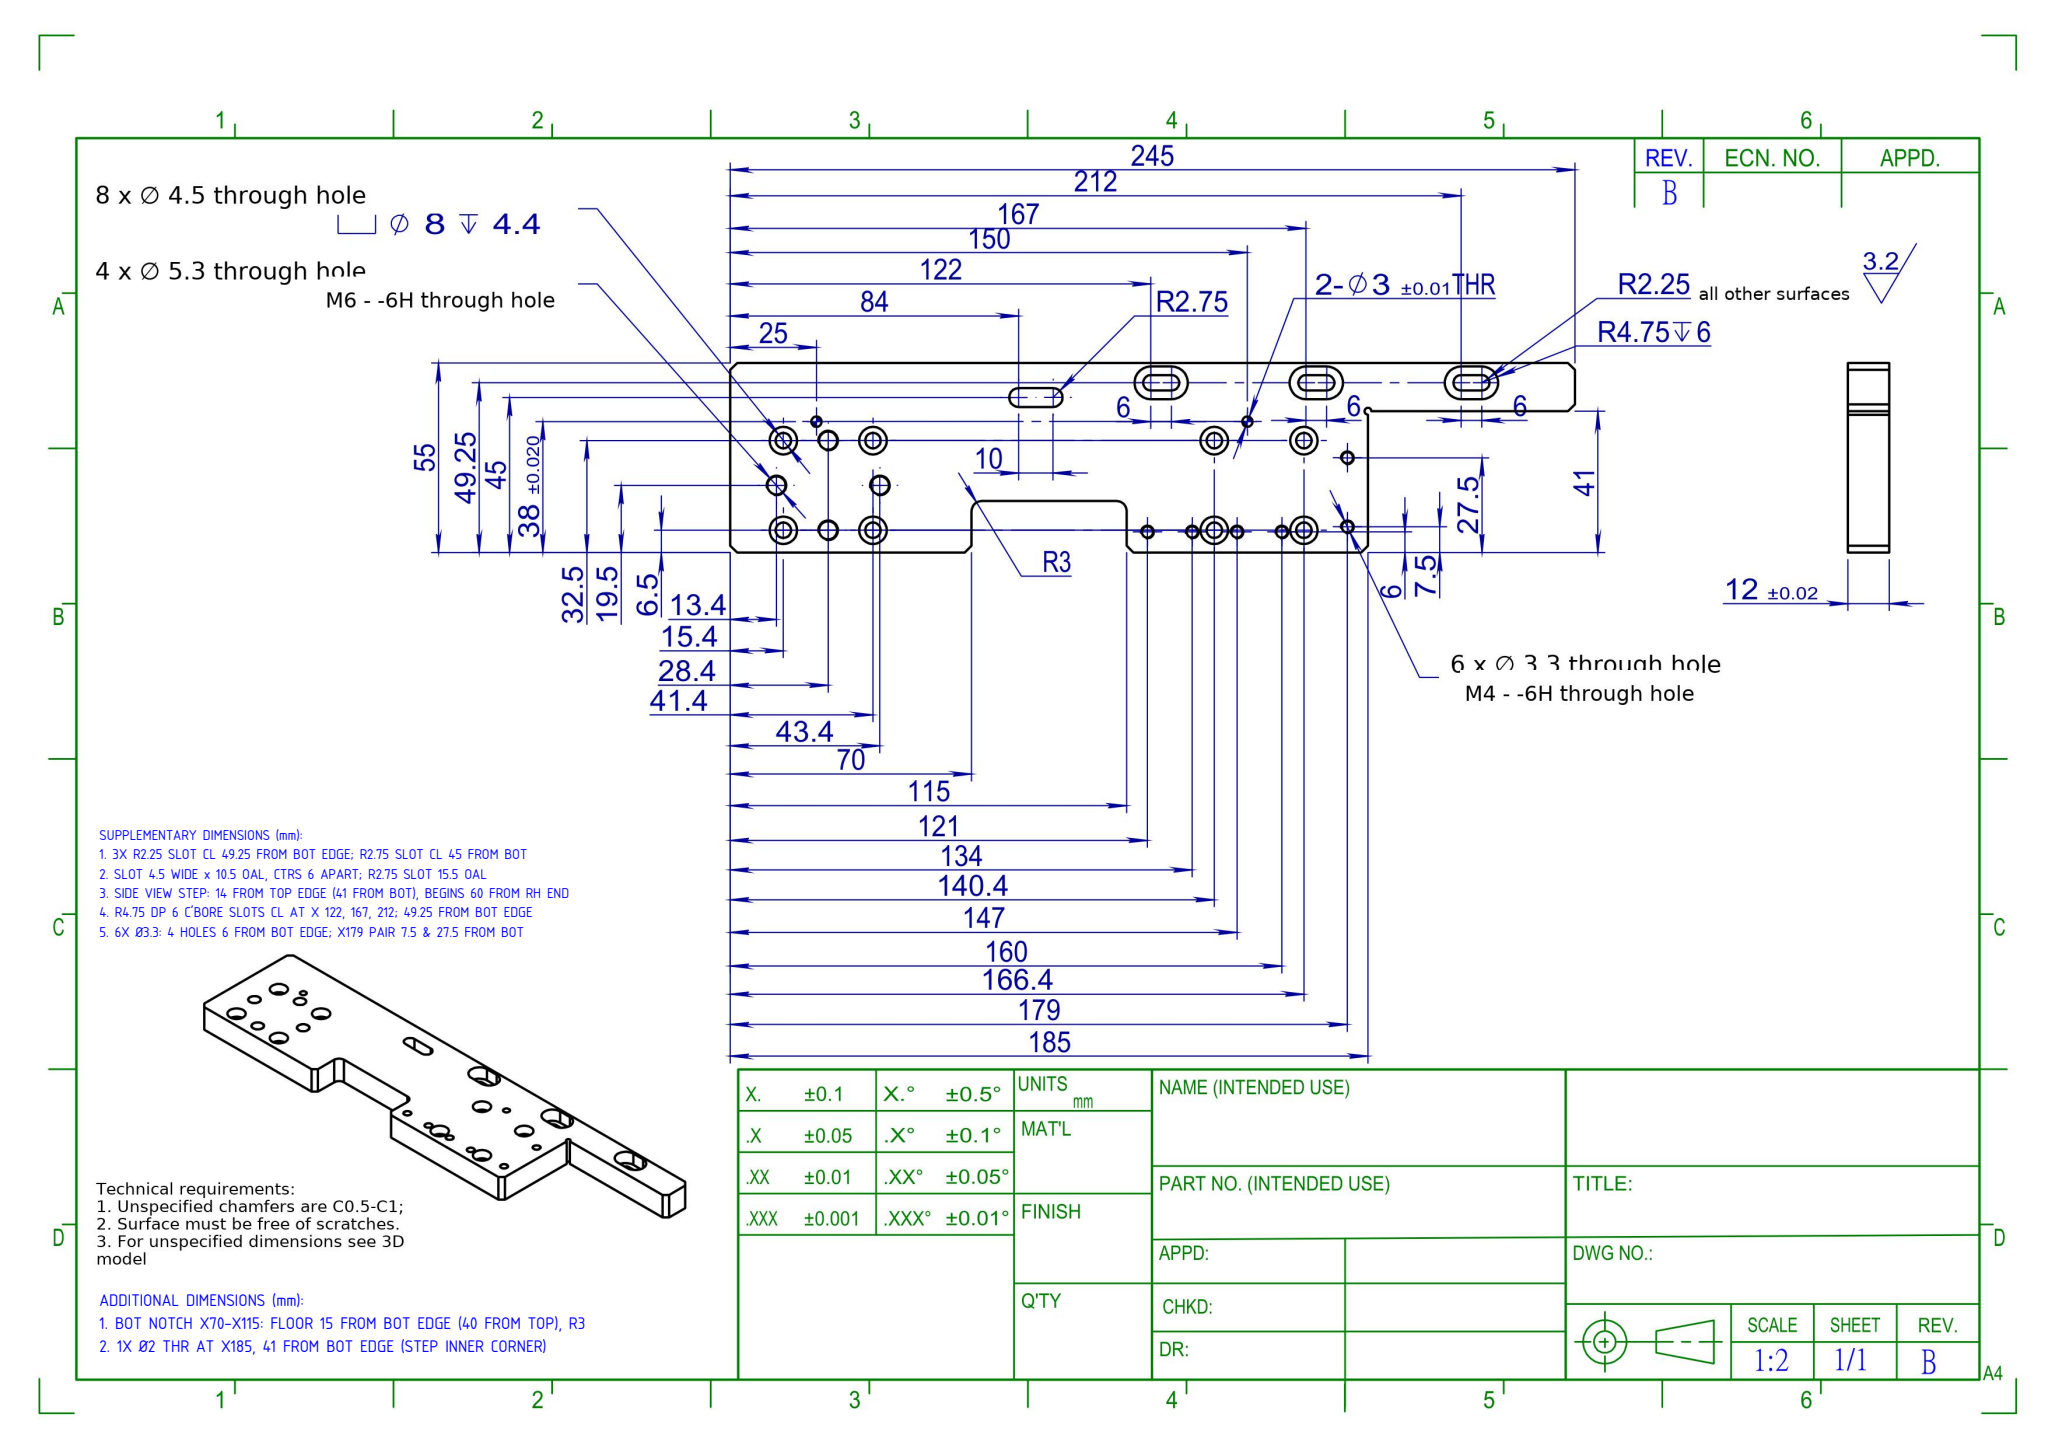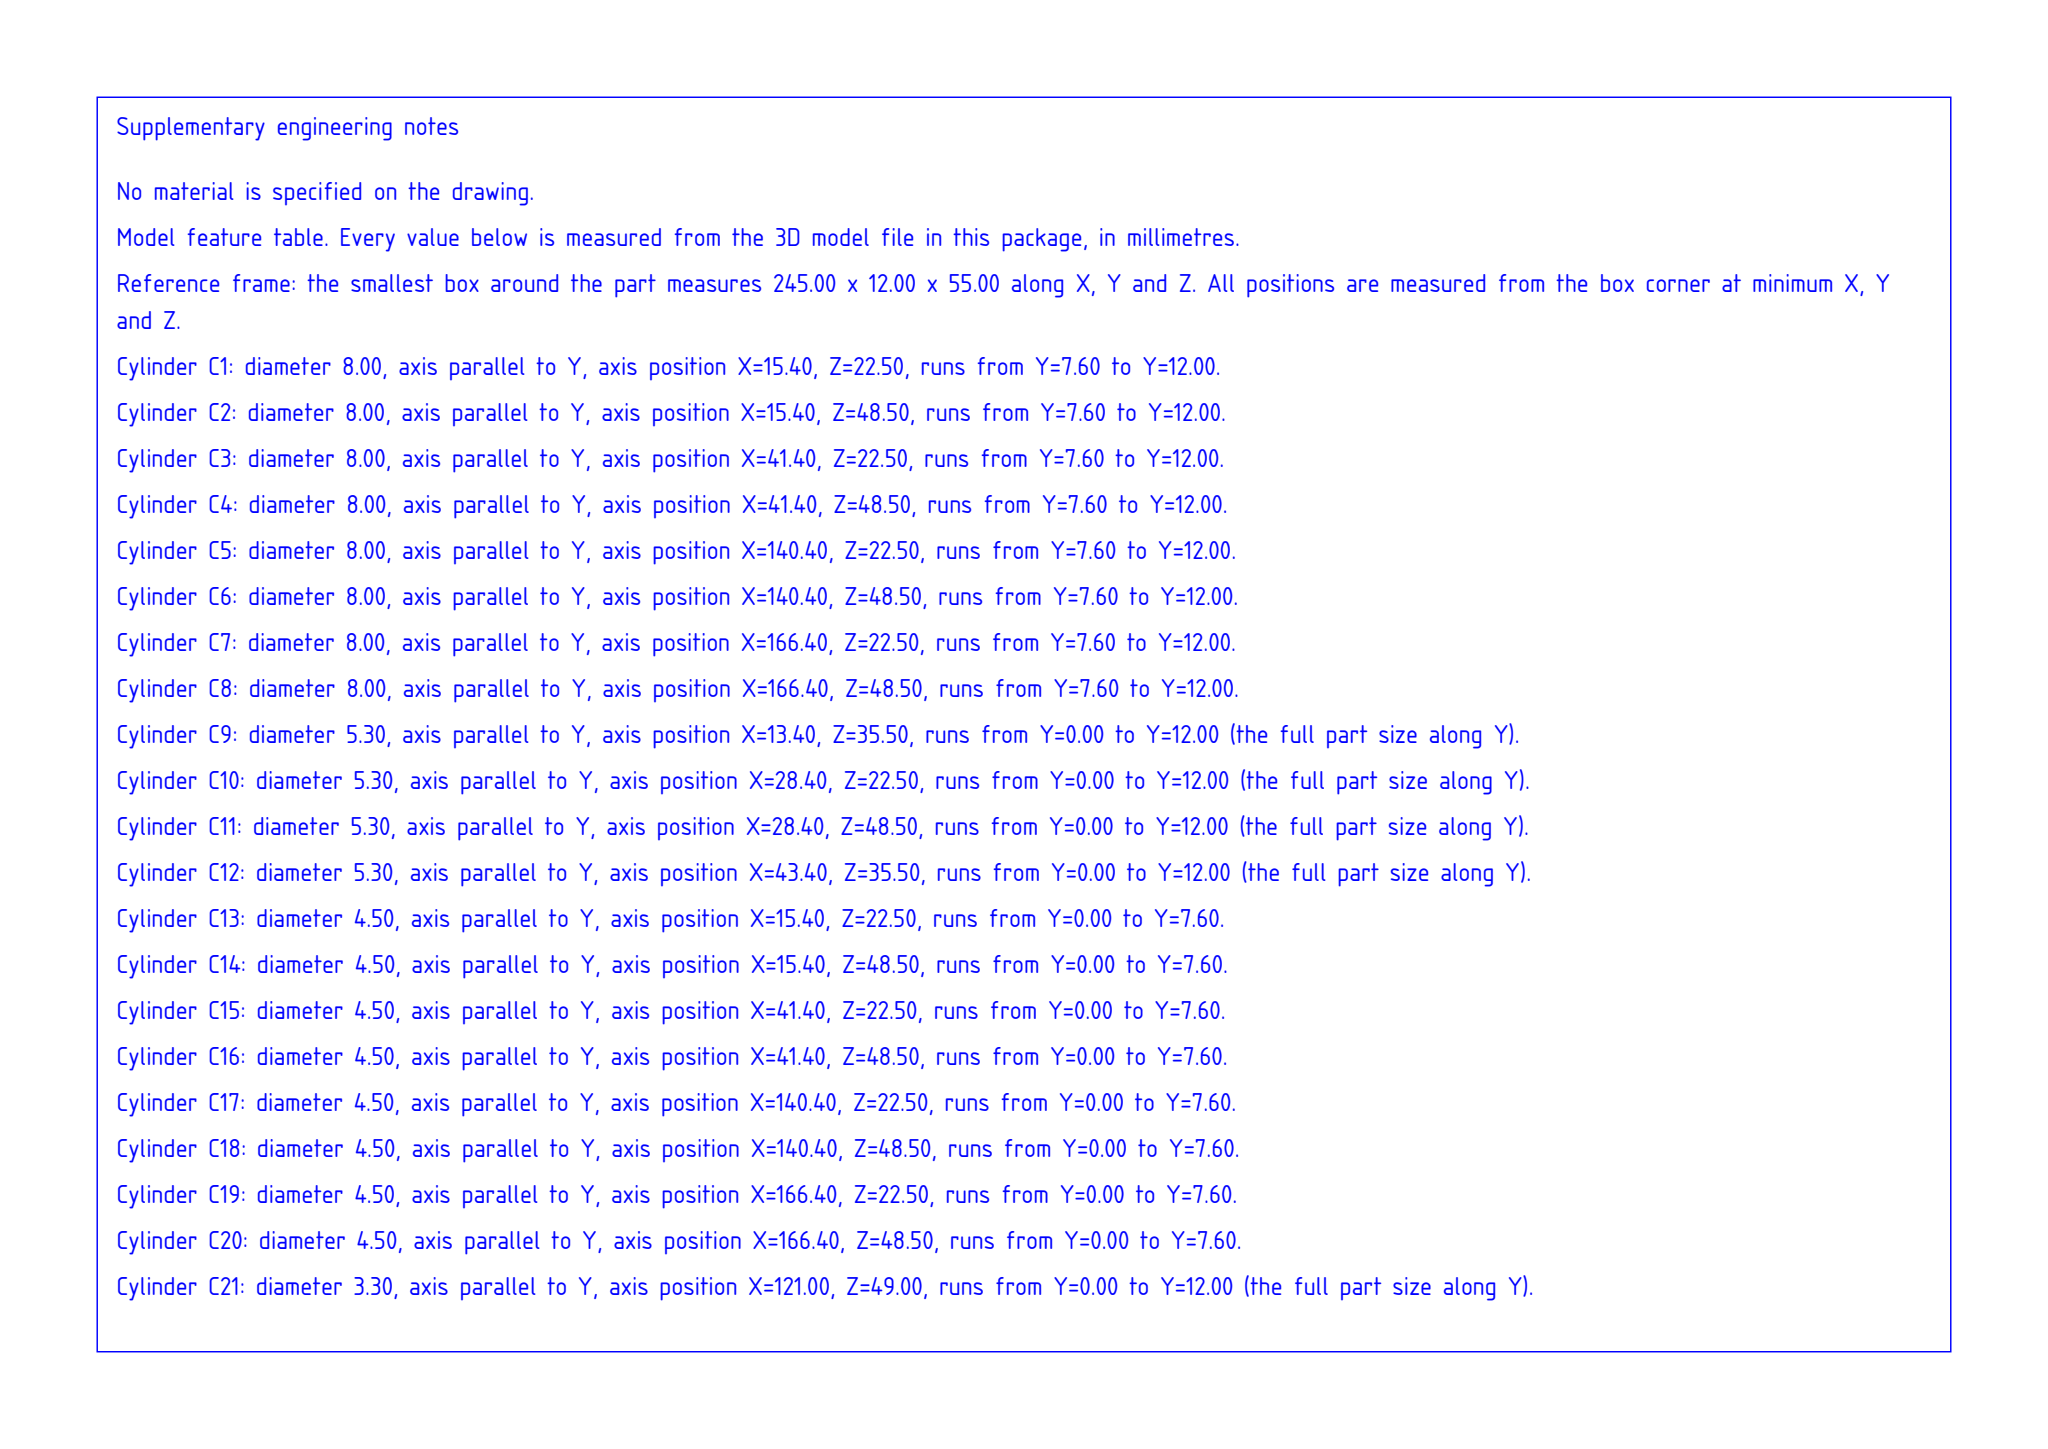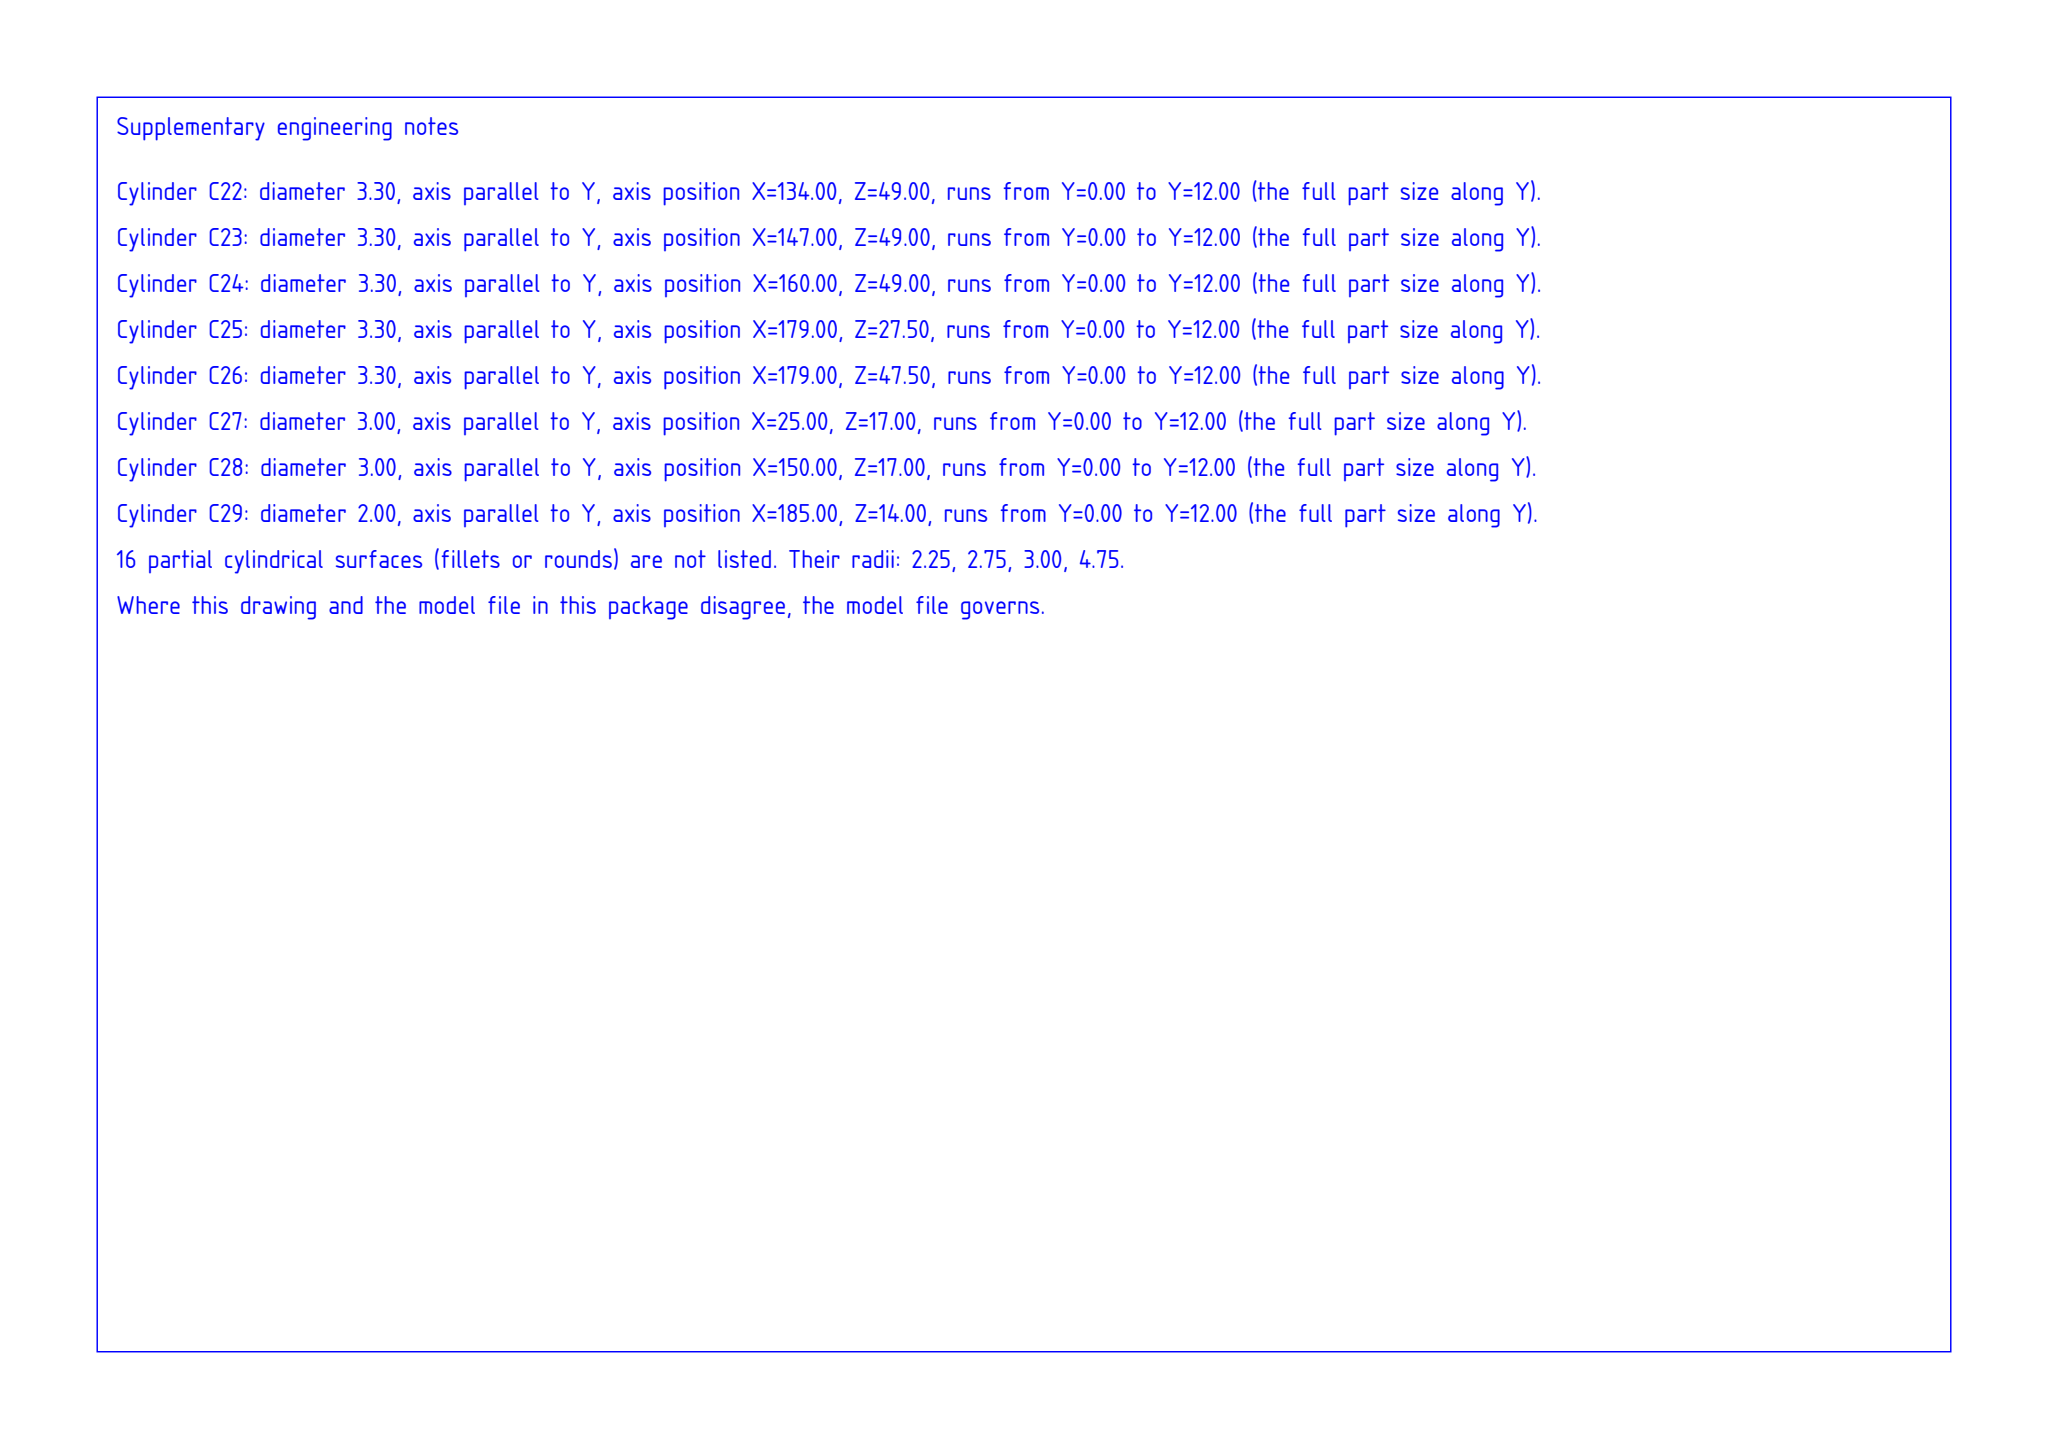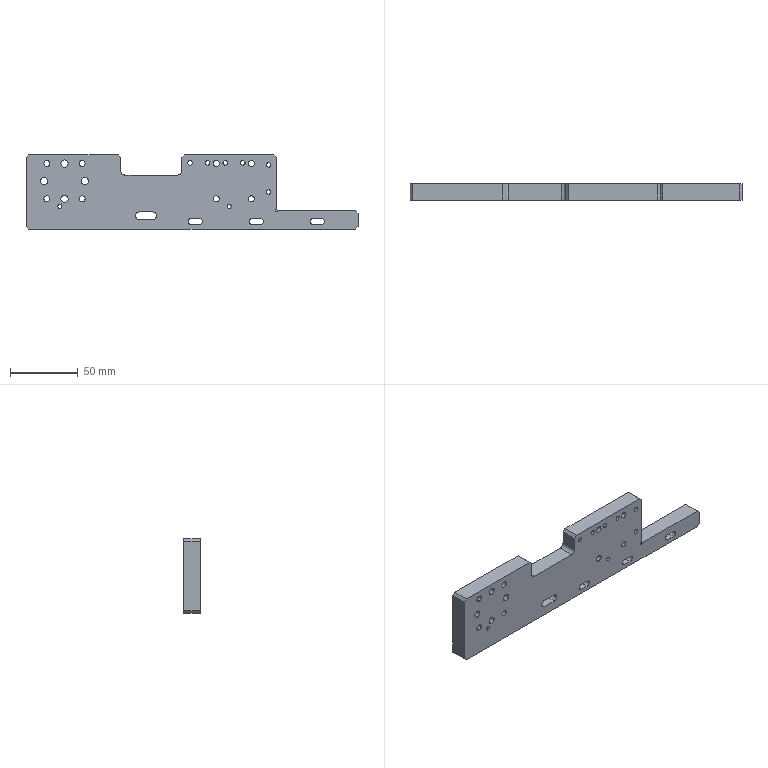Part | SolidWorks | mm | 1 solid | 117 faces | box 245 x 12 x 55 mm | volume 115330 mm3 | cylinder 73 | plane 44 | commonest cylinder face diameters 4.5 x22 8 x16 3.3 x12 5.3 x8 9.5 x6 3 x4 6 x2 5.5 x2
build123d program:
from build123d import *

# Parameters (mm, degrees)
SKETCH1_W                                            = 185
SKETCH1_H                                            = 165
BOSS_EXTRUDE1_DEPTH                                  = 12
SKETCH2_W                                            = 128
SKETCH2_H                                            = 110
CUT_EXTRUDE1_DEPTH                                   = 125.525
COUNTERBORE_FOR_M4_HEX_SOCKET_HEAD_CAP_S_D           = 4.5
COUNTERBORE_FOR_M4_HEX_SOCKET_HEAD_CAP_S_CBORE_D     = 8
COUNTERBORE_FOR_M4_HEX_SOCKET_HEAD_CAP_S_CBORE_DEPTH = 4.4
LINEAR_PATTERN1_COUNT                                = 2
LINEAR_PATTERN1_PITCH                                = 125
COUNTERBORE_FOR_M4_HEX_SOCKET_HEAD_C_2_D             = 4.5
COUNTERBORE_FOR_M4_HEX_SOCKET_HEAD_C_2_CBORE_D       = 8
COUNTERBORE_FOR_M4_HEX_SOCKET_HEAD_C_2_CBORE_DEPTH   = 4.4
SKETCH9_W                                            = 57
SKETCH9_H                                            = 30
CUT_EXTRUDE4_DEPTH                                   = 6.5
M4_TAPPED_HOLE1_D                                    = 3.3
CHAMFER1_SIZE                                        = 2
SKETCH24_W                                           = 62
SKETCH24_H                                           = 14
BOSS_EXTRUDE3_DEPTH                                  = 12
SKETCH17_W                                           = 45
SKETCH17_H                                           = 15
CUT_EXTRUDE8_DEPTH                                   = 174.8
FILLET3_R                                            = 3
CHAMFER2_SIZE                                        = 2
M4_TAPPED_HOLE2_D                                    = 3.3
BOSS_EXTRUDE2_REACH                                  = 175.8
SKETCH22_W                                           = 15
SKETCH22_H                                           = 45
SKETCH27_W                                           = 72
SKETCH27_H                                           = 110
CUT_EXTRUDE11_DEPTH                                  = 174.8
CHAMFER3_SIZE                                        = 2
CUT_EXTRUDE12_DEPTH                                  = 174.8
CUT_EXTRUDE13_DEPTH                                  = 6
LINEAR_PATTERN2_COUNT                                = 3
LINEAR_PATTERN2_PITCH                                = 45
SKETCH29_R                                           = 1.5
CUT_EXTRUDE14_DEPTH                                  = 174.8
M6_TAPPED_HOLE1_D                                    = 5.3
CUT_EXTRUDE15_DEPTH                                  = 174.8
SKETCH33_R                                           = 1
CUT_EXTRUDE16_DEPTH                                  = 174.8
CHAMFER4_SIZE                                        = 2


with BuildPart() as part:
    # Sketch1 → Boss-Extrude1 (new body)
    with BuildSketch(Plane(origin=(0, 0, 0), x_dir=(1, 0, 0), z_dir=(0, 1, 0))):
        Rectangle(SKETCH1_W, SKETCH1_H)
    extrude(amount=BOSS_EXTRUDE1_DEPTH)

    # Sketch2 → Cut-Extrude1 (cut, through all)
    with BuildSketch(Plane(origin=(0, 12, 0), x_dir=(1, 0, 0), z_dir=(0, 1, 0))):
        with Locations((28.5, 27.5)):
            Rectangle(SKETCH2_W, SKETCH2_H)
    extrude(amount=-CUT_EXTRUDE1_DEPTH, mode=Mode.SUBTRACT)

    # Counterbore for M4 Hex Socket Head Cap S (through all)
    with Locations(Plane(origin=(0, 12, 0), x_dir=(1, 0, 0), z_dir=(0, 1, 0))):
        with Locations((47.9, -76), (47.9, -50), (73.9, -50), (73.9, -76)):
            counterbore_for_m4_hex_socket_head_cap_s = CounterBoreHole(COUNTERBORE_FOR_M4_HEX_SOCKET_HEAD_CAP_S_D / 2, COUNTERBORE_FOR_M4_HEX_SOCKET_HEAD_CAP_S_CBORE_D / 2, COUNTERBORE_FOR_M4_HEX_SOCKET_HEAD_CAP_S_CBORE_DEPTH)

    # Linear Pattern1: Counterbore for M4 Hex Socket Head Cap S ×2
    with Locations(*[(-i * LINEAR_PATTERN1_PITCH, 0, 0) for i in range(1, LINEAR_PATTERN1_COUNT)]):
        add(counterbore_for_m4_hex_socket_head_cap_s, mode=Mode.SUBTRACT)

    # Counterbore for M4 Hex Socket Head C 2 (through all)
    with Locations(Plane(origin=(0, 12, 0), x_dir=(1, 0, 0), z_dir=(0, 1, 0))):
        with Locations((-77.1, 76), (-77.1, 50)):
            CounterBoreHole(COUNTERBORE_FOR_M4_HEX_SOCKET_HEAD_C_2_D / 2, COUNTERBORE_FOR_M4_HEX_SOCKET_HEAD_C_2_CBORE_D / 2, COUNTERBORE_FOR_M4_HEX_SOCKET_HEAD_C_2_CBORE_DEPTH)

    # Sketch9 → Cut-Extrude4 (cut)
    with BuildSketch(Plane.XZ):
        with Locations((-64, -31.5)):
            Rectangle(SKETCH9_W, SKETCH9_H)
    extrude(amount=-CUT_EXTRUDE4_DEPTH, mode=Mode.SUBTRACT)

    # M4 Tapped Hole1 (through all)
    with Locations(Plane(origin=(0, 12, 0), x_dir=(1, 0, 0), z_dir=(0, 1, 0))):
        with Locations((86.5, -75), (86.5, -55)):
            Hole(M4_TAPPED_HOLE1_D / 2)

    # Chamfer1
    chamfer1_edges = [part.edges().sort_by_distance(p)[0] for p in [
        (-35.5, 6, -82.5),
        (92.5, 6, 27.5),
        (-92.5, 6, -82.5),
        (92.5, 6, 82.5),
        (-92.5, 6, 82.5),
    ]]
    chamfer(chamfer1_edges, length=CHAMFER1_SIZE)

    # Sketch24 → Boss-Extrude3 (add)
    with BuildSketch(Plane.XZ):
        with Locations((121.5, 34.5)):
            Rectangle(SKETCH24_W, SKETCH24_H)
    extrude(amount=-BOSS_EXTRUDE3_DEPTH)

    # Sketch17 → Cut-Extrude8 (cut, through all)
    with BuildSketch(Plane(origin=(0, 12, 0), x_dir=(1, 0, 0), z_dir=(0, 1, 0))):
        with Locations((0, -75)):
            Rectangle(SKETCH17_W, SKETCH17_H)
    extrude(amount=-CUT_EXTRUDE8_DEPTH, mode=Mode.SUBTRACT)

    # Fillet3
    fillet3_edges = [part.edges().sort_by_distance(p)[0] for p in [
        (-22.5, 6, 67.5),
        (22.5, 6, 67.5),
    ]]
    fillet(fillet3_edges, radius=FILLET3_R)

    # Chamfer2
    chamfer2_edges = [part.edges().sort_by_distance(p)[0] for p in [
        (-22.5, 6, 82.5),
        (22.5, 6, 82.5),
    ]]
    chamfer(chamfer2_edges, length=CHAMFER2_SIZE)

    # M4 Tapped Hole2 (through all)
    with Locations(Plane(origin=(0, 12, 0), x_dir=(1, 0, 0), z_dir=(0, 1, 0))):
        with Locations((28.5, -76.5), (41.5, -76.5), (54.5, -76.5), (67.5, -76.5)):
            Hole(M4_TAPPED_HOLE2_D / 2)

    # Boss-Extrude2: up to this face of the body (flat: up to its plane)
    boss_extrude2_end = Plane(part.part.faces().sort_by_distance((-63.793, 0, -64.489))[0])
    # Sketch22 → Boss-Extrude2 (add, up to the picked face)
    with BuildSketch(Plane(origin=(0, 12, 0), x_dir=(1, 0, 0), z_dir=(0, 1, 0)), mode=Mode.PRIVATE) as boss_extrude2_sk1:
        with Locations((-28, -5)):
            Rectangle(SKETCH22_W, SKETCH22_H)
    boss_extrude2_tool1 = split(extrude(boss_extrude2_sk1.sketch, amount=-BOSS_EXTRUDE2_REACH, mode=Mode.PRIVATE), bisect_by=boss_extrude2_end, keep=Keep.BOTH, mode=Mode.PRIVATE)
    add(boss_extrude2_tool1.solids().sort_by(Axis((-28, 12, 5), (0, -1, 0)))[0])

    # Sketch27 → Cut-Extrude11 (cut, through all)
    with BuildSketch(Plane(origin=(0, 12, 0), x_dir=(1, 0, 0), z_dir=(0, 1, 0))):
        with Locations((-56.5, 27.5)):
            Rectangle(SKETCH27_W, SKETCH27_H)
    extrude(amount=-CUT_EXTRUDE11_DEPTH, mode=Mode.SUBTRACT)

    # Chamfer3
    chamfer3_edges = [part.edges().sort_by_distance(p)[0] for p in [
        (-92.5, 6, 27.5),
    ]]
    chamfer(chamfer3_edges, length=CHAMFER3_SIZE)

    # Sketch10 → Cut-Extrude12 (cut, through all)
    with BuildSketch(Plane(origin=(0, 12, 0), x_dir=(1, 0, 0), z_dir=(0, 1, 0))):
        with BuildLine():
            Line((125.5, -35.5), (119.5, -35.5))
            ThreePointArc((119.5, -35.5), (117.25, -33.25), (119.5, -31))
            Line((119.5, -31), (125.5, -31))
            ThreePointArc((125.5, -31), (127.75, -33.25), (125.5, -35.5))
        make_face()
    cut_extrude12 = extrude(amount=-CUT_EXTRUDE12_DEPTH, mode=Mode.SUBTRACT)

    # Sketch28 → Cut-Extrude13 (cut)
    with BuildSketch(Plane(origin=(0, 12, 0), x_dir=(1, 0, 0), z_dir=(0, 1, 0))):
        with BuildLine():
            Line((119.5, -38), (125.5, -38))
            ThreePointArc((125.5, -38), (130.25, -33.25), (125.5, -28.5))
            Line((125.5, -28.5), (119.5, -28.5))
            ThreePointArc((119.5, -28.5), (114.75, -33.25), (119.5, -38))
        make_face()
    cut_extrude13 = extrude(amount=-CUT_EXTRUDE13_DEPTH, mode=Mode.SUBTRACT)

    # Linear Pattern2: Cut-Extrude12, Cut-Extrude13 ×3
    with Locations(*[(-i * LINEAR_PATTERN2_PITCH, 0, 0) for i in range(1, LINEAR_PATTERN2_COUNT)]):
        add(cut_extrude12, mode=Mode.SUBTRACT)
        add(cut_extrude13, mode=Mode.SUBTRACT)

    # Sketch29 → Cut-Extrude14 (cut, through all)
    with BuildSketch(Plane(origin=(0, 12, 0), x_dir=(1, 0, 0), z_dir=(0, 1, 0))):
        with Locations(Location((-67.5, -44.5, 0), (0, 0, 270))):
            Circle(SKETCH29_R)
        with Locations(Location((57.5, -44.5, 0), (0, 0, 270))):
            Circle(SKETCH29_R)
    extrude(amount=-CUT_EXTRUDE14_DEPTH, mode=Mode.SUBTRACT)

    # M6 Tapped Hole1 (through all)
    with Locations(Plane(origin=(0, 12, 0), x_dir=(1, 0, 0), z_dir=(0, 1, 0))):
        with Locations((-49.1, -63), (-64.1, -50), (-79.1, -63), (-64.1, -76)):
            Hole(M6_TAPPED_HOLE1_D / 2)

    # Sketch32 → Cut-Extrude15 (cut, through all)
    with BuildSketch(Plane(origin=(0, 12, 0), x_dir=(1, 0, 0), z_dir=(0, 1, 0))):
        with BuildLine():
            Line((-8.854, -34.75), (1.146, -34.75))
            ThreePointArc((1.146, -34.75), (3.896, -37.5), (1.146, -40.25))
            Line((1.146, -40.25), (-8.854, -40.25))
            ThreePointArc((-8.854, -40.25), (-11.604, -37.5), (-8.854, -34.75))
        make_face()
    extrude(amount=-CUT_EXTRUDE15_DEPTH, mode=Mode.SUBTRACT)

    # Sketch33 → Cut-Extrude16 (cut, through all)
    with BuildSketch(Plane(origin=(0, 12, 0), x_dir=(1, 0, 0), z_dir=(0, 1, 0))):
        with Locations((92.5, -41.5)):
            Circle(SKETCH33_R)
    extrude(amount=-CUT_EXTRUDE16_DEPTH, mode=Mode.SUBTRACT)

    # Chamfer4
    chamfer4_edges = [part.edges().sort_by_distance(p)[0] for p in [
        (152.5, 6, 41.5),
        (152.5, 6, 27.5),
    ]]
    chamfer(chamfer4_edges, length=CHAMFER4_SIZE)


solid = part.part